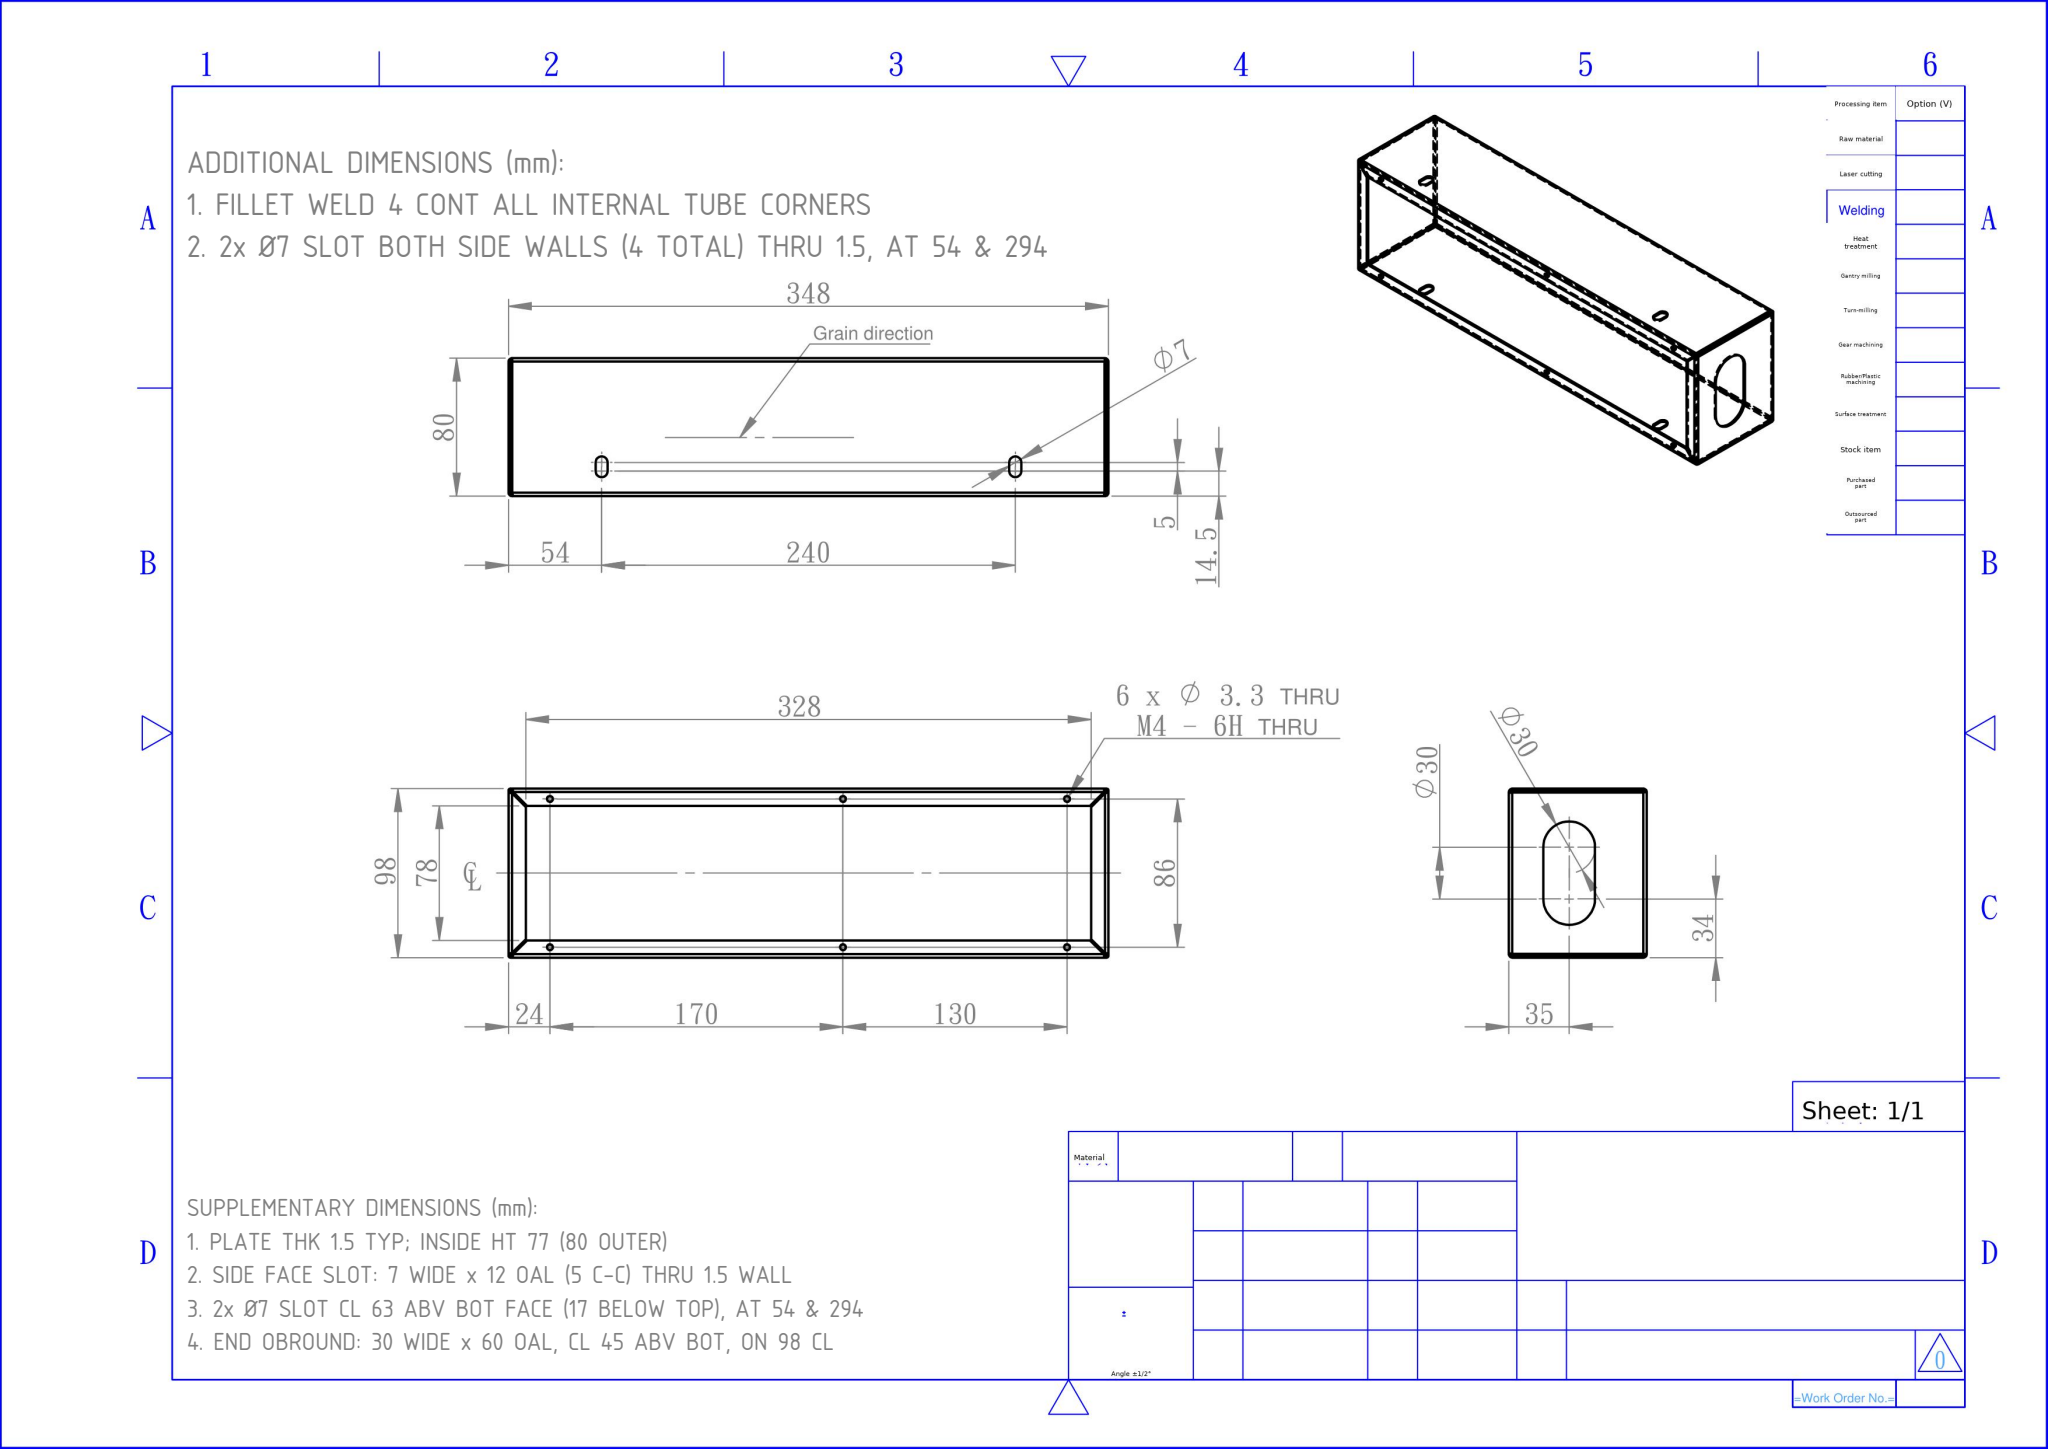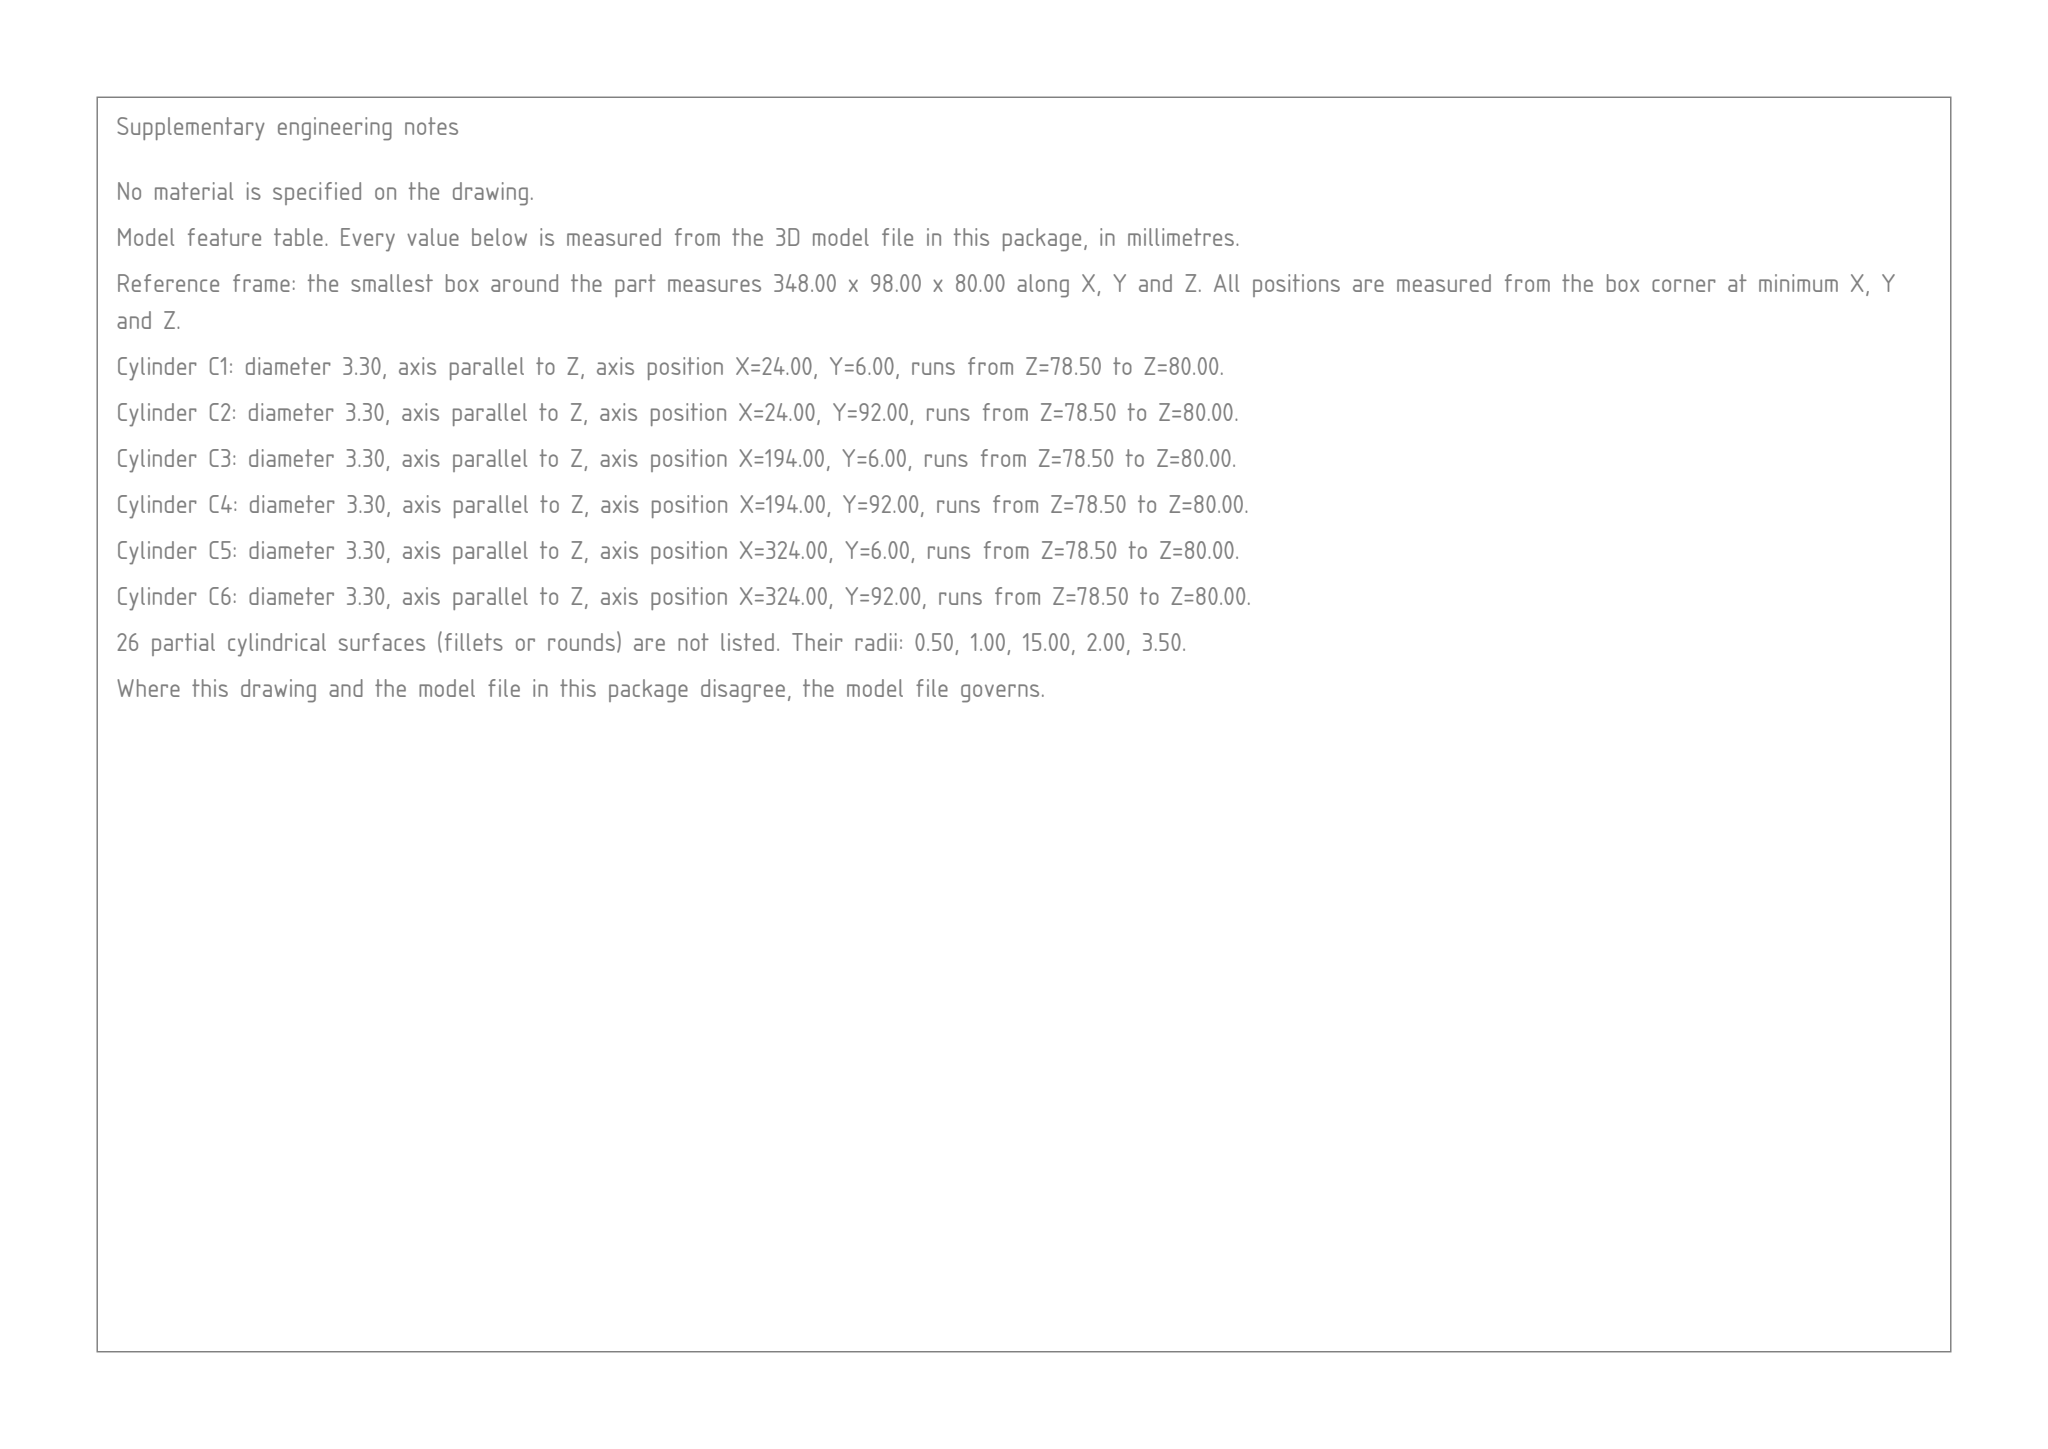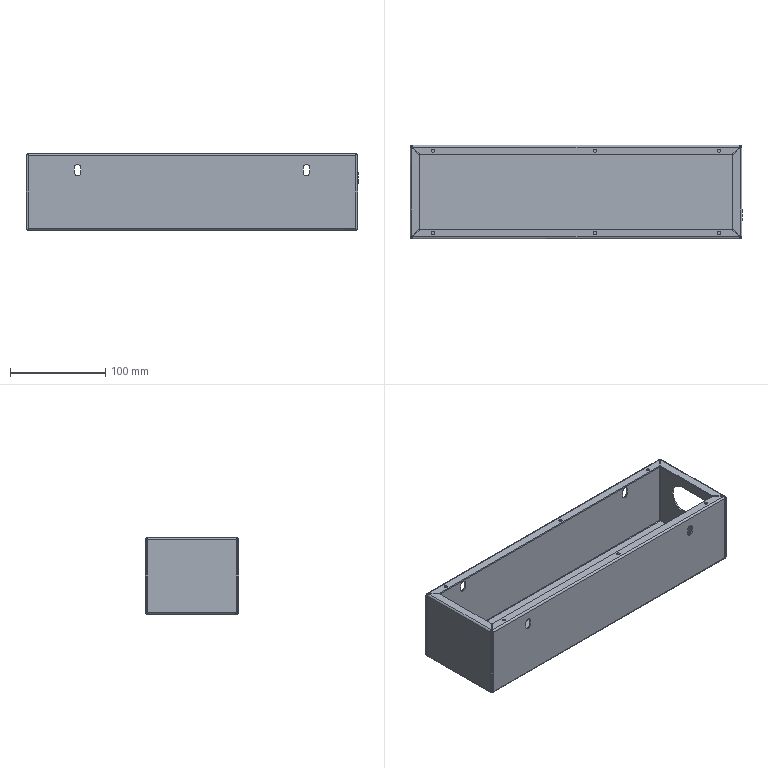Part | SolidWorks | mm | 1 solid | 150 faces | box 348 x 98 x 80 mm | volume 161844 mm3 | plane 64 | cylinder 46 | spline 40 | commonest cylinder face diameters 7 x12 3.3 x12 4 x8 1 x8 2 x4 30 x2